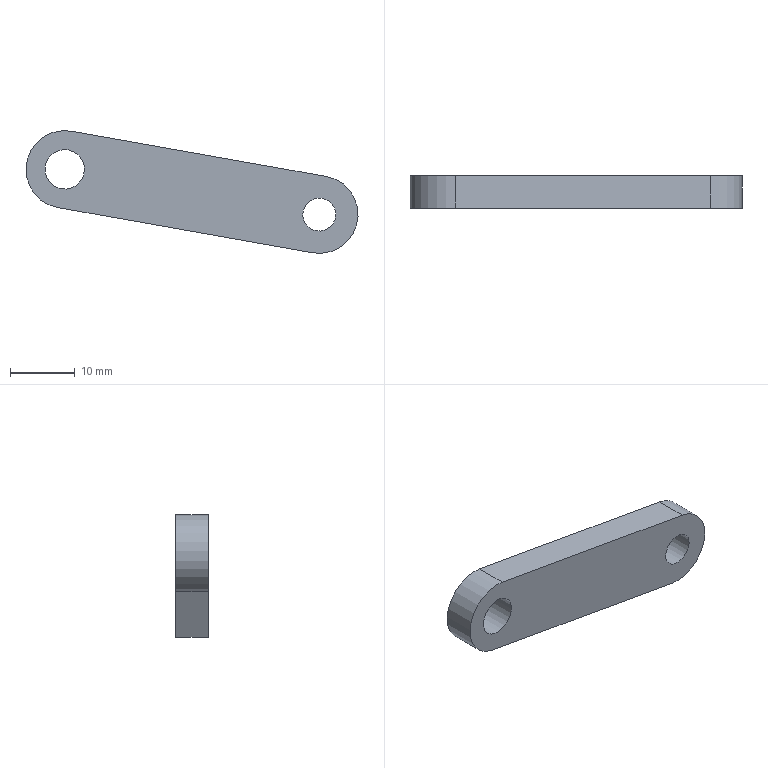Component | NX | LONG_LINK | 1 solid | 8 faces | box 51.38 x 5 x 19 mm | volume 2717 mm3 | plane 4 | cylinder 4 | commonest cylinder face diameters 12 x2 6.1 x1 5.1 x1
STEP:
#1=CARTESIAN_POINT('',(0.,0.,0.));
#2=DIRECTION('',(0.,0.,1.));
#3=DIRECTION('',(1.,0.,0.));
#4=AXIS2_PLACEMENT_3D('',#1,#2,#3);
#5=CARTESIAN_POINT('',(0.4327,-1.5,101.407));
#6=VERTEX_POINT('',#5);
#7=CARTESIAN_POINT('',(-38.95,-1.5,108.407));
#8=VERTEX_POINT('',#7);
#9=CARTESIAN_POINT('',(0.4327,-1.5,101.407));
#10=DIRECTION('',(-0.9846,0.,0.175));
#11=VECTOR('',#10,1.);
#12=LINE('',#9,#11);
#13=CARTESIAN_POINT('',(0.4327,-6.5,101.407));
#14=DIRECTION('',(-0.175,0.,-0.9846));
#15=DIRECTION('',(0.,-1.,0.));
#16=AXIS2_PLACEMENT_3D('',#13,#14,#15);
#17=PLANE('',#16);
#18=CARTESIAN_POINT('',(-5.,0.));
#19=DIRECTION('',(0.,1.));
#20=VECTOR('',#19,1.);
#21=LINE('',#18,#20);
#22=(GEOMETRIC_REPRESENTATION_CONTEXT(2)PARAMETRIC_REPRESENTATION_CONTEXT()REPRESENTATION_CONTEXT('',''));
#23=DEFINITIONAL_REPRESENTATION('',(#21),#22);
#24=PCURVE('',#17,#23);
#25=CARTESIAN_POINT('',(-40.,-1.5,102.5));
#26=DIRECTION('',(0.,-1.,0.));
#27=DIRECTION('',(0.175,0.,0.9846));
#28=AXIS2_PLACEMENT_3D('',#25,#26,#27);
#29=PLANE('',#28);
#30=CARTESIAN_POINT('',(6.,-40.));
#31=DIRECTION('',(0.,1.));
#32=VECTOR('',#31,1.);
#33=LINE('',#30,#32);
#34=(GEOMETRIC_REPRESENTATION_CONTEXT(2)PARAMETRIC_REPRESENTATION_CONTEXT()REPRESENTATION_CONTEXT('',''));
#35=DEFINITIONAL_REPRESENTATION('',(#33),#34);
#36=PCURVE('',#29,#35);
#37=SURFACE_CURVE('',#12,(#24,#36),.PCURVE_S1.);
#38=EDGE_CURVE('',#6,#8,#37,.T.);
#39=ORIENTED_EDGE('',*,*,#38,.T.);
#40=CARTESIAN_POINT('',(-38.95,-6.5,108.407));
#41=VERTEX_POINT('',#40);
#42=CARTESIAN_POINT('',(-38.95,-6.5,108.407));
#43=DIRECTION('',(0.,1.,0.));
#44=VECTOR('',#43,1.);
#45=LINE('',#42,#44);
#46=CARTESIAN_POINT('',(0.,40.));
#47=DIRECTION('',(-1.,0.));
#48=VECTOR('',#47,1.);
#49=LINE('',#46,#48);
#50=(GEOMETRIC_REPRESENTATION_CONTEXT(2)PARAMETRIC_REPRESENTATION_CONTEXT()REPRESENTATION_CONTEXT('',''));
#51=DEFINITIONAL_REPRESENTATION('',(#49),#50);
#52=PCURVE('',#17,#51);
#53=CARTESIAN_POINT('',(-40.,-6.5,102.5));
#54=DIRECTION('',(0.,1.,0.));
#55=DIRECTION('',(-0.175,0.,-0.9846));
#56=AXIS2_PLACEMENT_3D('',#53,#54,#55);
#57=CYLINDRICAL_SURFACE('',#56,6.);
#58=CARTESIAN_POINT('',(3.142,0.));
#59=DIRECTION('',(0.,1.));
#60=VECTOR('',#59,1.);
#61=LINE('',#58,#60);
#62=(GEOMETRIC_REPRESENTATION_CONTEXT(2)PARAMETRIC_REPRESENTATION_CONTEXT()REPRESENTATION_CONTEXT('',''));
#63=DEFINITIONAL_REPRESENTATION('',(#61),#62);
#64=PCURVE('',#57,#63);
#65=SURFACE_CURVE('',#45,(#52,#64),.PCURVE_S1.);
#66=EDGE_CURVE('',#41,#8,#65,.T.);
#67=ORIENTED_EDGE('',*,*,#66,.F.);
#68=CARTESIAN_POINT('',(0.4327,-6.5,101.407));
#69=VERTEX_POINT('',#68);
#70=CARTESIAN_POINT('',(0.4327,-6.5,101.407));
#71=DIRECTION('',(-0.9846,0.,0.175));
#72=VECTOR('',#71,1.);
#73=LINE('',#70,#72);
#74=CARTESIAN_POINT('',(0.,0.));
#75=DIRECTION('',(0.,1.));
#76=VECTOR('',#75,1.);
#77=LINE('',#74,#76);
#78=(GEOMETRIC_REPRESENTATION_CONTEXT(2)PARAMETRIC_REPRESENTATION_CONTEXT()REPRESENTATION_CONTEXT('',''));
#79=DEFINITIONAL_REPRESENTATION('',(#77),#78);
#80=PCURVE('',#17,#79);
#81=CARTESIAN_POINT('',(-40.,-6.5,102.5));
#82=DIRECTION('',(0.,-1.,0.));
#83=DIRECTION('',(0.175,0.,0.9846));
#84=AXIS2_PLACEMENT_3D('',#81,#82,#83);
#85=PLANE('',#84);
#86=CARTESIAN_POINT('',(6.,-40.));
#87=DIRECTION('',(0.,1.));
#88=VECTOR('',#87,1.);
#89=LINE('',#86,#88);
#90=(GEOMETRIC_REPRESENTATION_CONTEXT(2)PARAMETRIC_REPRESENTATION_CONTEXT()REPRESENTATION_CONTEXT('',''));
#91=DEFINITIONAL_REPRESENTATION('',(#89),#90);
#92=PCURVE('',#85,#91);
#93=SURFACE_CURVE('',#73,(#80,#92),.PCURVE_S1.);
#94=EDGE_CURVE('',#69,#41,#93,.T.);
#95=ORIENTED_EDGE('',*,*,#94,.F.);
#96=CARTESIAN_POINT('',(0.4327,-6.5,101.407));
#97=DIRECTION('',(0.,1.,0.));
#98=VECTOR('',#97,1.);
#99=LINE('',#96,#98);
#100=CARTESIAN_POINT('',(0.,0.));
#101=DIRECTION('',(-1.,0.));
#102=VECTOR('',#101,1.);
#103=LINE('',#100,#102);
#104=(GEOMETRIC_REPRESENTATION_CONTEXT(2)PARAMETRIC_REPRESENTATION_CONTEXT()REPRESENTATION_CONTEXT('',''));
#105=DEFINITIONAL_REPRESENTATION('',(#103),#104);
#106=PCURVE('',#17,#105);
#107=CARTESIAN_POINT('',(-0.6173,-6.5,95.5));
#108=DIRECTION('',(0.,1.,0.));
#109=DIRECTION('',(-0.175,0.,-0.9846));
#110=AXIS2_PLACEMENT_3D('',#107,#108,#109);
#111=CYLINDRICAL_SURFACE('',#110,6.);
#112=CARTESIAN_POINT('',(3.142,0.));
#113=DIRECTION('',(0.,1.));
#114=VECTOR('',#113,1.);
#115=LINE('',#112,#114);
#116=(GEOMETRIC_REPRESENTATION_CONTEXT(2)PARAMETRIC_REPRESENTATION_CONTEXT()REPRESENTATION_CONTEXT('',''));
#117=DEFINITIONAL_REPRESENTATION('',(#115),#116);
#118=PCURVE('',#111,#117);
#119=SURFACE_CURVE('',#99,(#106,#118),.PCURVE_S1.);
#120=EDGE_CURVE('',#69,#6,#119,.T.);
#121=ORIENTED_EDGE('',*,*,#120,.T.);
#122=EDGE_LOOP('',(#39,#67,#95,#121));
#123=FACE_BOUND('',#122,.T.);
#124=ADVANCED_FACE('',(#123),#17,.F.);
#125=CARTESIAN_POINT('',(-41.05,-1.5,96.593));
#126=VERTEX_POINT('',#125);
#127=CARTESIAN_POINT('',(-40.,-1.5,102.5));
#128=DIRECTION('',(0.,-1.,0.));
#129=DIRECTION('',(0.175,0.,0.9846));
#130=AXIS2_PLACEMENT_3D('',#127,#128,#129);
#131=CIRCLE('',#130,6.);
#132=CARTESIAN_POINT('',(3.142,5.));
#133=DIRECTION('',(-1.,0.));
#134=VECTOR('',#133,1.);
#135=LINE('',#132,#134);
#136=(GEOMETRIC_REPRESENTATION_CONTEXT(2)PARAMETRIC_REPRESENTATION_CONTEXT()REPRESENTATION_CONTEXT('',''));
#137=DEFINITIONAL_REPRESENTATION('',(#135),#136);
#138=PCURVE('',#57,#137);
#139=CARTESIAN_POINT('',(0.,0.));
#140=DIRECTION('',(1.,0.));
#141=AXIS2_PLACEMENT_2D('',#139,#140);
#142=CIRCLE('',#141,6.);
#143=(GEOMETRIC_REPRESENTATION_CONTEXT(2)PARAMETRIC_REPRESENTATION_CONTEXT()REPRESENTATION_CONTEXT('',''));
#144=DEFINITIONAL_REPRESENTATION('',(#142),#143);
#145=PCURVE('',#29,#144);
#146=SURFACE_CURVE('',#131,(#138,#145),.PCURVE_S1.);
#147=EDGE_CURVE('',#8,#126,#146,.T.);
#148=ORIENTED_EDGE('',*,*,#147,.T.);
#149=CARTESIAN_POINT('',(-41.05,-6.5,96.593));
#150=VERTEX_POINT('',#149);
#151=CARTESIAN_POINT('',(-41.05,-6.5,96.593));
#152=DIRECTION('',(0.,1.,0.));
#153=VECTOR('',#152,1.);
#154=LINE('',#151,#153);
#155=CARTESIAN_POINT('',(0.,0.));
#156=DIRECTION('',(0.,1.));
#157=VECTOR('',#156,1.);
#158=LINE('',#155,#157);
#159=(GEOMETRIC_REPRESENTATION_CONTEXT(2)PARAMETRIC_REPRESENTATION_CONTEXT()REPRESENTATION_CONTEXT('',''));
#160=DEFINITIONAL_REPRESENTATION('',(#158),#159);
#161=PCURVE('',#57,#160);
#162=CARTESIAN_POINT('',(-41.05,-6.5,96.593));
#163=DIRECTION('',(0.175,0.,0.9846));
#164=DIRECTION('',(0.,1.,0.));
#165=AXIS2_PLACEMENT_3D('',#162,#163,#164);
#166=PLANE('',#165);
#167=CARTESIAN_POINT('',(0.,0.));
#168=DIRECTION('',(1.,0.));
#169=VECTOR('',#168,1.);
#170=LINE('',#167,#169);
#171=(GEOMETRIC_REPRESENTATION_CONTEXT(2)PARAMETRIC_REPRESENTATION_CONTEXT()REPRESENTATION_CONTEXT('',''));
#172=DEFINITIONAL_REPRESENTATION('',(#170),#171);
#173=PCURVE('',#166,#172);
#174=SURFACE_CURVE('',#154,(#161,#173),.PCURVE_S1.);
#175=EDGE_CURVE('',#150,#126,#174,.T.);
#176=ORIENTED_EDGE('',*,*,#175,.F.);
#177=CARTESIAN_POINT('',(-40.,-6.5,102.5));
#178=DIRECTION('',(0.,-1.,0.));
#179=DIRECTION('',(0.175,0.,0.9846));
#180=AXIS2_PLACEMENT_3D('',#177,#178,#179);
#181=CIRCLE('',#180,6.);
#182=CARTESIAN_POINT('',(3.142,0.));
#183=DIRECTION('',(-1.,0.));
#184=VECTOR('',#183,1.);
#185=LINE('',#182,#184);
#186=(GEOMETRIC_REPRESENTATION_CONTEXT(2)PARAMETRIC_REPRESENTATION_CONTEXT()REPRESENTATION_CONTEXT('',''));
#187=DEFINITIONAL_REPRESENTATION('',(#185),#186);
#188=PCURVE('',#57,#187);
#189=CARTESIAN_POINT('',(0.,0.));
#190=DIRECTION('',(1.,0.));
#191=AXIS2_PLACEMENT_2D('',#189,#190);
#192=CIRCLE('',#191,6.);
#193=(GEOMETRIC_REPRESENTATION_CONTEXT(2)PARAMETRIC_REPRESENTATION_CONTEXT()REPRESENTATION_CONTEXT('',''));
#194=DEFINITIONAL_REPRESENTATION('',(#192),#193);
#195=PCURVE('',#85,#194);
#196=SURFACE_CURVE('',#181,(#188,#195),.PCURVE_S1.);
#197=EDGE_CURVE('',#41,#150,#196,.T.);
#198=ORIENTED_EDGE('',*,*,#197,.F.);
#199=ORIENTED_EDGE('',*,*,#66,.T.);
#200=EDGE_LOOP('',(#148,#176,#198,#199));
#201=FACE_BOUND('',#200,.T.);
#202=ADVANCED_FACE('',(#201),#57,.T.);
#203=CARTESIAN_POINT('',(-1.667,-1.5,89.593));
#204=VERTEX_POINT('',#203);
#205=CARTESIAN_POINT('',(-41.05,-1.5,96.593));
#206=DIRECTION('',(0.9846,0.,-0.175));
#207=VECTOR('',#206,1.);
#208=LINE('',#205,#207);
#209=CARTESIAN_POINT('',(5.,0.));
#210=DIRECTION('',(0.,-1.));
#211=VECTOR('',#210,1.);
#212=LINE('',#209,#211);
#213=(GEOMETRIC_REPRESENTATION_CONTEXT(2)PARAMETRIC_REPRESENTATION_CONTEXT()REPRESENTATION_CONTEXT('',''));
#214=DEFINITIONAL_REPRESENTATION('',(#212),#213);
#215=PCURVE('',#166,#214);
#216=CARTESIAN_POINT('',(-6.,-0.));
#217=DIRECTION('',(0.,-1.));
#218=VECTOR('',#217,1.);
#219=LINE('',#216,#218);
#220=(GEOMETRIC_REPRESENTATION_CONTEXT(2)PARAMETRIC_REPRESENTATION_CONTEXT()REPRESENTATION_CONTEXT('',''));
#221=DEFINITIONAL_REPRESENTATION('',(#219),#220);
#222=PCURVE('',#29,#221);
#223=SURFACE_CURVE('',#208,(#215,#222),.PCURVE_S1.);
#224=EDGE_CURVE('',#126,#204,#223,.T.);
#225=ORIENTED_EDGE('',*,*,#224,.T.);
#226=CARTESIAN_POINT('',(-1.667,-6.5,89.593));
#227=VERTEX_POINT('',#226);
#228=CARTESIAN_POINT('',(-1.667,-6.5,89.593));
#229=DIRECTION('',(0.,1.,0.));
#230=VECTOR('',#229,1.);
#231=LINE('',#228,#230);
#232=CARTESIAN_POINT('',(0.,-40.));
#233=DIRECTION('',(1.,0.));
#234=VECTOR('',#233,1.);
#235=LINE('',#232,#234);
#236=(GEOMETRIC_REPRESENTATION_CONTEXT(2)PARAMETRIC_REPRESENTATION_CONTEXT()REPRESENTATION_CONTEXT('',''));
#237=DEFINITIONAL_REPRESENTATION('',(#235),#236);
#238=PCURVE('',#166,#237);
#239=CARTESIAN_POINT('',(6.283,0.));
#240=DIRECTION('',(0.,1.));
#241=VECTOR('',#240,1.);
#242=LINE('',#239,#241);
#243=(GEOMETRIC_REPRESENTATION_CONTEXT(2)PARAMETRIC_REPRESENTATION_CONTEXT()REPRESENTATION_CONTEXT('',''));
#244=DEFINITIONAL_REPRESENTATION('',(#242),#243);
#245=PCURVE('',#111,#244);
#246=SURFACE_CURVE('',#231,(#238,#245),.PCURVE_S1.);
#247=EDGE_CURVE('',#227,#204,#246,.T.);
#248=ORIENTED_EDGE('',*,*,#247,.F.);
#249=CARTESIAN_POINT('',(-41.05,-6.5,96.593));
#250=DIRECTION('',(0.9846,0.,-0.175));
#251=VECTOR('',#250,1.);
#252=LINE('',#249,#251);
#253=CARTESIAN_POINT('',(0.,0.));
#254=DIRECTION('',(0.,-1.));
#255=VECTOR('',#254,1.);
#256=LINE('',#253,#255);
#257=(GEOMETRIC_REPRESENTATION_CONTEXT(2)PARAMETRIC_REPRESENTATION_CONTEXT()REPRESENTATION_CONTEXT('',''));
#258=DEFINITIONAL_REPRESENTATION('',(#256),#257);
#259=PCURVE('',#166,#258);
#260=CARTESIAN_POINT('',(-6.,-0.));
#261=DIRECTION('',(0.,-1.));
#262=VECTOR('',#261,1.);
#263=LINE('',#260,#262);
#264=(GEOMETRIC_REPRESENTATION_CONTEXT(2)PARAMETRIC_REPRESENTATION_CONTEXT()REPRESENTATION_CONTEXT('',''));
#265=DEFINITIONAL_REPRESENTATION('',(#263),#264);
#266=PCURVE('',#85,#265);
#267=SURFACE_CURVE('',#252,(#259,#266),.PCURVE_S1.);
#268=EDGE_CURVE('',#150,#227,#267,.T.);
#269=ORIENTED_EDGE('',*,*,#268,.F.);
#270=ORIENTED_EDGE('',*,*,#175,.T.);
#271=EDGE_LOOP('',(#225,#248,#269,#270));
#272=FACE_BOUND('',#271,.T.);
#273=ADVANCED_FACE('',(#272),#166,.F.);
#274=CARTESIAN_POINT('',(-39.466,-6.5,105.503));
#275=VERTEX_POINT('',#274);
#276=CARTESIAN_POINT('',(-40.,-6.5,102.5));
#277=DIRECTION('',(0.,-1.,0.));
#278=DIRECTION('',(0.175,0.,0.9846));
#279=AXIS2_PLACEMENT_3D('',#276,#277,#278);
#280=CIRCLE('',#279,3.05);
#281=CARTESIAN_POINT('',(-40.,-6.5,102.5));
#282=DIRECTION('',(0.,1.,0.));
#283=DIRECTION('',(-0.175,0.,-0.9846));
#284=AXIS2_PLACEMENT_3D('',#281,#282,#283);
#285=CYLINDRICAL_SURFACE('',#284,3.05);
#286=CARTESIAN_POINT('',(9.425,0.));
#287=DIRECTION('',(-1.,0.));
#288=VECTOR('',#287,1.);
#289=LINE('',#286,#288);
#290=(GEOMETRIC_REPRESENTATION_CONTEXT(2)PARAMETRIC_REPRESENTATION_CONTEXT()REPRESENTATION_CONTEXT('',''));
#291=DEFINITIONAL_REPRESENTATION('',(#289),#290);
#292=PCURVE('',#285,#291);
#293=CARTESIAN_POINT('',(0.,0.));
#294=DIRECTION('',(1.,-0.));
#295=AXIS2_PLACEMENT_2D('',#293,#294);
#296=CIRCLE('',#295,3.05);
#297=(GEOMETRIC_REPRESENTATION_CONTEXT(2)PARAMETRIC_REPRESENTATION_CONTEXT()REPRESENTATION_CONTEXT('',''));
#298=DEFINITIONAL_REPRESENTATION('',(#296),#297);
#299=PCURVE('',#85,#298);
#300=SURFACE_CURVE('',#280,(#292,#299),.PCURVE_S1.);
#301=EDGE_CURVE('',#275,#275,#300,.T.);
#302=ORIENTED_EDGE('',*,*,#301,.F.);
#303=CARTESIAN_POINT('',(-39.466,-1.5,105.503));
#304=VERTEX_POINT('',#303);
#305=CARTESIAN_POINT('',(-39.466,-6.5,105.503));
#306=CARTESIAN_POINT('',(-39.466,-1.5,105.503));
#307=B_SPLINE_CURVE_WITH_KNOTS('',1,(#305,#306),.UNSPECIFIED.,.F.,.F.,(2,2),(0.,5.),.PIECEWISE_BEZIER_KNOTS.);
#308=CARTESIAN_POINT('',(9.425,0.));
#309=DIRECTION('',(0.,1.));
#310=VECTOR('',#309,1.);
#311=LINE('',#308,#310);
#312=(GEOMETRIC_REPRESENTATION_CONTEXT(2)PARAMETRIC_REPRESENTATION_CONTEXT()REPRESENTATION_CONTEXT('',''));
#313=DEFINITIONAL_REPRESENTATION('',(#311),#312);
#314=PCURVE('',#285,#313);
#315=CARTESIAN_POINT('',(3.142,0.));
#316=DIRECTION('',(0.,1.));
#317=VECTOR('',#316,1.);
#318=LINE('',#315,#317);
#319=(GEOMETRIC_REPRESENTATION_CONTEXT(2)PARAMETRIC_REPRESENTATION_CONTEXT()REPRESENTATION_CONTEXT('',''));
#320=DEFINITIONAL_REPRESENTATION('',(#318),#319);
#321=PCURVE('',#285,#320);
#322=SEAM_CURVE('',#307,(#314,#321),.PCURVE_S1.);
#323=EDGE_CURVE('',#275,#304,#322,.T.);
#324=ORIENTED_EDGE('',*,*,#323,.T.);
#325=CARTESIAN_POINT('',(-40.,-1.5,102.5));
#326=DIRECTION('',(0.,-1.,0.));
#327=DIRECTION('',(0.175,0.,0.9846));
#328=AXIS2_PLACEMENT_3D('',#325,#326,#327);
#329=CIRCLE('',#328,3.05);
#330=CARTESIAN_POINT('',(9.425,5.));
#331=DIRECTION('',(-1.,0.));
#332=VECTOR('',#331,1.);
#333=LINE('',#330,#332);
#334=(GEOMETRIC_REPRESENTATION_CONTEXT(2)PARAMETRIC_REPRESENTATION_CONTEXT()REPRESENTATION_CONTEXT('',''));
#335=DEFINITIONAL_REPRESENTATION('',(#333),#334);
#336=PCURVE('',#285,#335);
#337=CARTESIAN_POINT('',(0.,0.));
#338=DIRECTION('',(1.,-0.));
#339=AXIS2_PLACEMENT_2D('',#337,#338);
#340=CIRCLE('',#339,3.05);
#341=(GEOMETRIC_REPRESENTATION_CONTEXT(2)PARAMETRIC_REPRESENTATION_CONTEXT()REPRESENTATION_CONTEXT('',''));
#342=DEFINITIONAL_REPRESENTATION('',(#340),#341);
#343=PCURVE('',#29,#342);
#344=SURFACE_CURVE('',#329,(#336,#343),.PCURVE_S1.);
#345=EDGE_CURVE('',#304,#304,#344,.T.);
#346=ORIENTED_EDGE('',*,*,#345,.T.);
#347=ORIENTED_EDGE('',*,*,#323,.F.);
#348=EDGE_LOOP('',(#302,#324,#346,#347));
#349=FACE_BOUND('',#348,.F.);
#350=ADVANCED_FACE('',(#349),#285,.F.);
#351=CARTESIAN_POINT('',(-0.6173,-1.5,95.5));
#352=DIRECTION('',(0.,-1.,0.));
#353=DIRECTION('',(0.175,0.,0.9846));
#354=AXIS2_PLACEMENT_3D('',#351,#352,#353);
#355=CIRCLE('',#354,6.);
#356=CARTESIAN_POINT('',(9.425,5.));
#357=DIRECTION('',(-1.,0.));
#358=VECTOR('',#357,1.);
#359=LINE('',#356,#358);
#360=(GEOMETRIC_REPRESENTATION_CONTEXT(2)PARAMETRIC_REPRESENTATION_CONTEXT()REPRESENTATION_CONTEXT('',''));
#361=DEFINITIONAL_REPRESENTATION('',(#359),#360);
#362=PCURVE('',#111,#361);
#363=CARTESIAN_POINT('',(0.,-40.));
#364=DIRECTION('',(1.,0.));
#365=AXIS2_PLACEMENT_2D('',#363,#364);
#366=CIRCLE('',#365,6.);
#367=(GEOMETRIC_REPRESENTATION_CONTEXT(2)PARAMETRIC_REPRESENTATION_CONTEXT()REPRESENTATION_CONTEXT('',''));
#368=DEFINITIONAL_REPRESENTATION('',(#366),#367);
#369=PCURVE('',#29,#368);
#370=SURFACE_CURVE('',#355,(#362,#369),.PCURVE_S1.);
#371=EDGE_CURVE('',#204,#6,#370,.T.);
#372=ORIENTED_EDGE('',*,*,#371,.T.);
#373=ORIENTED_EDGE('',*,*,#120,.F.);
#374=CARTESIAN_POINT('',(-0.6173,-6.5,95.5));
#375=DIRECTION('',(0.,-1.,0.));
#376=DIRECTION('',(0.175,0.,0.9846));
#377=AXIS2_PLACEMENT_3D('',#374,#375,#376);
#378=CIRCLE('',#377,6.);
#379=CARTESIAN_POINT('',(9.425,0.));
#380=DIRECTION('',(-1.,0.));
#381=VECTOR('',#380,1.);
#382=LINE('',#379,#381);
#383=(GEOMETRIC_REPRESENTATION_CONTEXT(2)PARAMETRIC_REPRESENTATION_CONTEXT()REPRESENTATION_CONTEXT('',''));
#384=DEFINITIONAL_REPRESENTATION('',(#382),#383);
#385=PCURVE('',#111,#384);
#386=CARTESIAN_POINT('',(0.,-40.));
#387=DIRECTION('',(1.,0.));
#388=AXIS2_PLACEMENT_2D('',#386,#387);
#389=CIRCLE('',#388,6.);
#390=(GEOMETRIC_REPRESENTATION_CONTEXT(2)PARAMETRIC_REPRESENTATION_CONTEXT()REPRESENTATION_CONTEXT('',''));
#391=DEFINITIONAL_REPRESENTATION('',(#389),#390);
#392=PCURVE('',#85,#391);
#393=SURFACE_CURVE('',#378,(#385,#392),.PCURVE_S1.);
#394=EDGE_CURVE('',#227,#69,#393,.T.);
#395=ORIENTED_EDGE('',*,*,#394,.F.);
#396=ORIENTED_EDGE('',*,*,#247,.T.);
#397=EDGE_LOOP('',(#372,#373,#395,#396));
#398=FACE_BOUND('',#397,.T.);
#399=ADVANCED_FACE('',(#398),#111,.T.);
#400=CARTESIAN_POINT('',(-0.171,-6.5,98.011));
#401=VERTEX_POINT('',#400);
#402=CARTESIAN_POINT('',(-0.6173,-6.5,95.5));
#403=DIRECTION('',(0.,-1.,0.));
#404=DIRECTION('',(0.175,0.,0.9846));
#405=AXIS2_PLACEMENT_3D('',#402,#403,#404);
#406=CIRCLE('',#405,2.55);
#407=CARTESIAN_POINT('',(-0.6173,-6.5,95.5));
#408=DIRECTION('',(0.,1.,0.));
#409=DIRECTION('',(-0.175,0.,-0.9846));
#410=AXIS2_PLACEMENT_3D('',#407,#408,#409);
#411=CYLINDRICAL_SURFACE('',#410,2.55);
#412=CARTESIAN_POINT('',(9.425,0.));
#413=DIRECTION('',(-1.,0.));
#414=VECTOR('',#413,1.);
#415=LINE('',#412,#414);
#416=(GEOMETRIC_REPRESENTATION_CONTEXT(2)PARAMETRIC_REPRESENTATION_CONTEXT()REPRESENTATION_CONTEXT('',''));
#417=DEFINITIONAL_REPRESENTATION('',(#415),#416);
#418=PCURVE('',#411,#417);
#419=CARTESIAN_POINT('',(0.,-40.));
#420=DIRECTION('',(1.,0.));
#421=AXIS2_PLACEMENT_2D('',#419,#420);
#422=CIRCLE('',#421,2.55);
#423=(GEOMETRIC_REPRESENTATION_CONTEXT(2)PARAMETRIC_REPRESENTATION_CONTEXT()REPRESENTATION_CONTEXT('',''));
#424=DEFINITIONAL_REPRESENTATION('',(#422),#423);
#425=PCURVE('',#85,#424);
#426=SURFACE_CURVE('',#406,(#418,#425),.PCURVE_S1.);
#427=EDGE_CURVE('',#401,#401,#426,.T.);
#428=ORIENTED_EDGE('',*,*,#427,.F.);
#429=CARTESIAN_POINT('',(-0.171,-1.5,98.011));
#430=VERTEX_POINT('',#429);
#431=CARTESIAN_POINT('',(-0.171,-6.5,98.011));
#432=CARTESIAN_POINT('',(-0.171,-1.5,98.011));
#433=B_SPLINE_CURVE_WITH_KNOTS('',1,(#431,#432),.UNSPECIFIED.,.F.,.F.,(2,2),(0.,5.),.PIECEWISE_BEZIER_KNOTS.);
#434=CARTESIAN_POINT('',(9.425,0.));
#435=DIRECTION('',(0.,1.));
#436=VECTOR('',#435,1.);
#437=LINE('',#434,#436);
#438=(GEOMETRIC_REPRESENTATION_CONTEXT(2)PARAMETRIC_REPRESENTATION_CONTEXT()REPRESENTATION_CONTEXT('',''));
#439=DEFINITIONAL_REPRESENTATION('',(#437),#438);
#440=PCURVE('',#411,#439);
#441=CARTESIAN_POINT('',(3.142,0.));
#442=DIRECTION('',(0.,1.));
#443=VECTOR('',#442,1.);
#444=LINE('',#441,#443);
#445=(GEOMETRIC_REPRESENTATION_CONTEXT(2)PARAMETRIC_REPRESENTATION_CONTEXT()REPRESENTATION_CONTEXT('',''));
#446=DEFINITIONAL_REPRESENTATION('',(#444),#445);
#447=PCURVE('',#411,#446);
#448=SEAM_CURVE('',#433,(#440,#447),.PCURVE_S1.);
#449=EDGE_CURVE('',#401,#430,#448,.T.);
#450=ORIENTED_EDGE('',*,*,#449,.T.);
#451=CARTESIAN_POINT('',(-0.6173,-1.5,95.5));
#452=DIRECTION('',(0.,-1.,0.));
#453=DIRECTION('',(0.175,0.,0.9846));
#454=AXIS2_PLACEMENT_3D('',#451,#452,#453);
#455=CIRCLE('',#454,2.55);
#456=CARTESIAN_POINT('',(9.425,5.));
#457=DIRECTION('',(-1.,0.));
#458=VECTOR('',#457,1.);
#459=LINE('',#456,#458);
#460=(GEOMETRIC_REPRESENTATION_CONTEXT(2)PARAMETRIC_REPRESENTATION_CONTEXT()REPRESENTATION_CONTEXT('',''));
#461=DEFINITIONAL_REPRESENTATION('',(#459),#460);
#462=PCURVE('',#411,#461);
#463=CARTESIAN_POINT('',(0.,-40.));
#464=DIRECTION('',(1.,0.));
#465=AXIS2_PLACEMENT_2D('',#463,#464);
#466=CIRCLE('',#465,2.55);
#467=(GEOMETRIC_REPRESENTATION_CONTEXT(2)PARAMETRIC_REPRESENTATION_CONTEXT()REPRESENTATION_CONTEXT('',''));
#468=DEFINITIONAL_REPRESENTATION('',(#466),#467);
#469=PCURVE('',#29,#468);
#470=SURFACE_CURVE('',#455,(#462,#469),.PCURVE_S1.);
#471=EDGE_CURVE('',#430,#430,#470,.T.);
#472=ORIENTED_EDGE('',*,*,#471,.T.);
#473=ORIENTED_EDGE('',*,*,#449,.F.);
#474=EDGE_LOOP('',(#428,#450,#472,#473));
#475=FACE_BOUND('',#474,.F.);
#476=ADVANCED_FACE('',(#475),#411,.F.);
#477=ORIENTED_EDGE('',*,*,#94,.T.);
#478=ORIENTED_EDGE('',*,*,#197,.T.);
#479=ORIENTED_EDGE('',*,*,#268,.T.);
#480=ORIENTED_EDGE('',*,*,#394,.T.);
#481=EDGE_LOOP('',(#477,#478,#479,#480));
#482=FACE_BOUND('',#481,.T.);
#483=ORIENTED_EDGE('',*,*,#301,.F.);
#484=EDGE_LOOP('',(#483));
#485=FACE_BOUND('',#484,.T.);
#486=ORIENTED_EDGE('',*,*,#427,.F.);
#487=EDGE_LOOP('',(#486));
#488=FACE_BOUND('',#487,.T.);
#489=ADVANCED_FACE('',(#482,#485,#488),#85,.T.);
#490=ORIENTED_EDGE('',*,*,#38,.F.);
#491=ORIENTED_EDGE('',*,*,#371,.F.);
#492=ORIENTED_EDGE('',*,*,#224,.F.);
#493=ORIENTED_EDGE('',*,*,#147,.F.);
#494=EDGE_LOOP('',(#490,#491,#492,#493));
#495=FACE_BOUND('',#494,.T.);
#496=ORIENTED_EDGE('',*,*,#345,.T.);
#497=EDGE_LOOP('',(#496));
#498=FACE_BOUND('',#497,.T.);
#499=ORIENTED_EDGE('',*,*,#471,.T.);
#500=EDGE_LOOP('',(#499));
#501=FACE_BOUND('',#500,.T.);
#502=ADVANCED_FACE('',(#495,#498,#501),#29,.F.);
#503=CLOSED_SHELL('',(#124,#202,#273,#350,#399,#476,#489,#502));
#504=MANIFOLD_SOLID_BREP('',#503);
#505=(LENGTH_UNIT()NAMED_UNIT(*)SI_UNIT(.MILLI.,.METRE.));
#506=UNCERTAINTY_MEASURE_WITH_UNIT(LENGTH_MEASURE(0.000002),#505,'','');
#507=(NAMED_UNIT(*)PLANE_ANGLE_UNIT()SI_UNIT($,.RADIAN.));
#508=(NAMED_UNIT(*)SI_UNIT($,.STERADIAN.)SOLID_ANGLE_UNIT());
#509=(GEOMETRIC_REPRESENTATION_CONTEXT(3)GLOBAL_UNCERTAINTY_ASSIGNED_CONTEXT((#506))GLOBAL_UNIT_ASSIGNED_CONTEXT((#505,#507,#508))REPRESENTATION_CONTEXT('',''));
#510=ADVANCED_BREP_SHAPE_REPRESENTATION('',(#4,#504),#509);